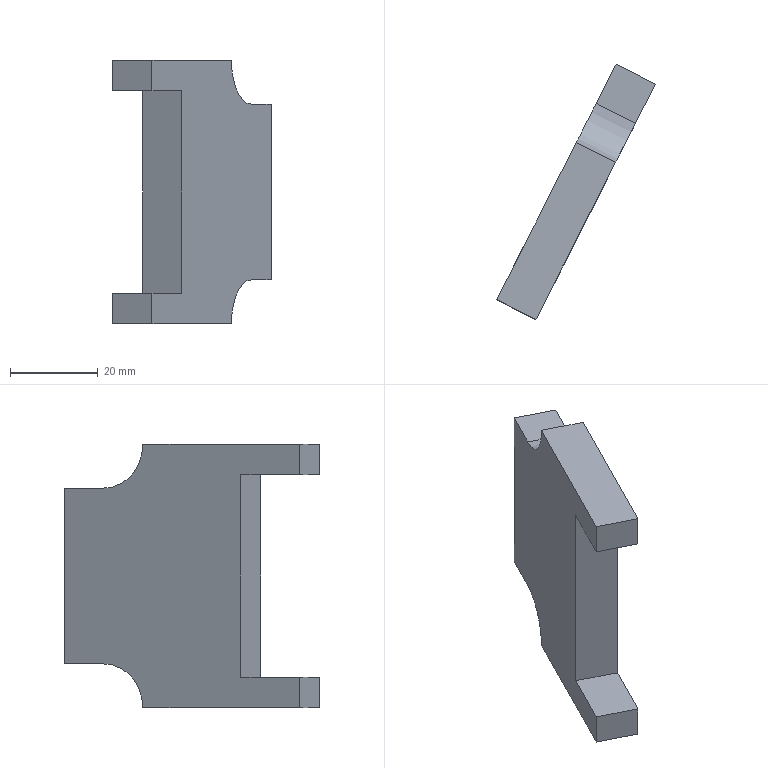Component | SolidWorks | PartThree-1 | 1 solid | 14 faces | box 36.05 x 58.04 x 60 mm | volume 25529 mm3 | plane 12 | cylinder 2 | commonest cylinder face diameters 20 x2
STEP:
#1=CARTESIAN_POINT('',(-56.846,-10.874,42.676));
#2=VERTEX_POINT('',#1);
#3=CARTESIAN_POINT('',(-56.495,-11.052,42.676));
#4=VERTEX_POINT('',#3);
#5=CARTESIAN_POINT('',(-56.846,-10.874,42.676));
#6=DIRECTION('',(0.892,-0.4521,-0.));
#7=VECTOR('',#6,39.37);
#8=LINE('',#5,#7);
#9=EDGE_CURVE('',#2,#4,#8,.T.);
#10=ORIENTED_EDGE('',*,*,#9,.F.);
#11=CARTESIAN_POINT('',(-57.024,-11.225,43.07));
#12=VERTEX_POINT('',#11);
#13=CARTESIAN_POINT('',(-56.846,-10.874,43.07));
#14=DIRECTION('',(-0.892,0.4521,0.));
#15=DIRECTION('',(-0.,-0.,1.));
#16=AXIS2_PLACEMENT_3D('',#13,#14,#15);
#17=CIRCLE('',#16,0.3937);
#18=EDGE_CURVE('',#2,#12,#17,.T.);
#19=ORIENTED_EDGE('',*,*,#18,.T.);
#20=CARTESIAN_POINT('',(-56.673,-11.403,43.07));
#21=VERTEX_POINT('',#20);
#22=CARTESIAN_POINT('',(-57.024,-11.225,43.07));
#23=DIRECTION('',(0.892,-0.4521,-0.));
#24=VECTOR('',#23,39.37);
#25=LINE('',#22,#24);
#26=EDGE_CURVE('',#12,#21,#25,.T.);
#27=ORIENTED_EDGE('',*,*,#26,.T.);
#28=CARTESIAN_POINT('',(-56.495,-11.052,43.07));
#29=DIRECTION('',(0.892,-0.4521,-0.));
#30=DIRECTION('',(-0.,-0.,1.));
#31=AXIS2_PLACEMENT_3D('',#28,#29,#30);
#32=CIRCLE('',#31,0.3937);
#33=EDGE_CURVE('',#21,#4,#32,.T.);
#34=ORIENTED_EDGE('',*,*,#33,.T.);
#35=EDGE_LOOP('',(#10,#19,#27,#34));
#36=FACE_OUTER_BOUND('',#35,.T.);
#37=CARTESIAN_POINT('',(-56.846,-10.874,43.07));
#38=DIRECTION('',(-0.892,0.4521,0.));
#39=DIRECTION('',(-0.,-0.,1.));
#40=AXIS2_PLACEMENT_3D('',#37,#38,#39);
#41=CYLINDRICAL_SURFACE('',#40,0.3937);
#42=ADVANCED_FACE('',(#36),#41,.F.);
#43=CARTESIAN_POINT('',(-56.495,-11.052,41.101));
#44=VERTEX_POINT('',#43);
#45=CARTESIAN_POINT('',(-56.846,-10.874,41.101));
#46=VERTEX_POINT('',#45);
#47=CARTESIAN_POINT('',(-56.846,-10.874,41.101));
#48=DIRECTION('',(-0.892,0.4521,0.));
#49=VECTOR('',#48,39.37);
#50=LINE('',#47,#49);
#51=EDGE_CURVE('',#44,#46,#50,.T.);
#52=ORIENTED_EDGE('',*,*,#51,.F.);
#53=CARTESIAN_POINT('',(-56.673,-11.403,40.708));
#54=VERTEX_POINT('',#53);
#55=CARTESIAN_POINT('',(-56.495,-11.052,40.708));
#56=DIRECTION('',(0.892,-0.4521,-0.));
#57=DIRECTION('',(-0.,-0.,1.));
#58=AXIS2_PLACEMENT_3D('',#55,#56,#57);
#59=CIRCLE('',#58,0.3937);
#60=EDGE_CURVE('',#44,#54,#59,.T.);
#61=ORIENTED_EDGE('',*,*,#60,.T.);
#62=CARTESIAN_POINT('',(-57.024,-11.225,40.708));
#63=VERTEX_POINT('',#62);
#64=CARTESIAN_POINT('',(-57.024,-11.225,40.708));
#65=DIRECTION('',(0.892,-0.4521,-0.));
#66=VECTOR('',#65,39.37);
#67=LINE('',#64,#66);
#68=EDGE_CURVE('',#63,#54,#67,.T.);
#69=ORIENTED_EDGE('',*,*,#68,.F.);
#70=CARTESIAN_POINT('',(-56.846,-10.874,40.708));
#71=DIRECTION('',(-0.892,0.4521,0.));
#72=DIRECTION('',(-0.,-0.,1.));
#73=AXIS2_PLACEMENT_3D('',#70,#71,#72);
#74=CIRCLE('',#73,0.3937);
#75=EDGE_CURVE('',#63,#46,#74,.T.);
#76=ORIENTED_EDGE('',*,*,#75,.T.);
#77=EDGE_LOOP('',(#52,#61,#69,#76));
#78=FACE_OUTER_BOUND('',#77,.T.);
#79=CARTESIAN_POINT('',(-56.846,-10.874,40.708));
#80=DIRECTION('',(0.892,-0.4521,-0.));
#81=DIRECTION('',(0.,0.,-1.));
#82=AXIS2_PLACEMENT_3D('',#79,#80,#81);
#83=CYLINDRICAL_SURFACE('',#82,0.3937);
#84=ADVANCED_FACE('',(#78),#83,.F.);
#85=CARTESIAN_POINT('',(-57.385,-12.808,40.708));
#86=VERTEX_POINT('',#85);
#87=CARTESIAN_POINT('',(-56.673,-11.403,40.708));
#88=DIRECTION('',(-0.4521,-0.892,-0.));
#89=VECTOR('',#88,39.37);
#90=LINE('',#87,#89);
#91=EDGE_CURVE('',#54,#86,#90,.T.);
#92=ORIENTED_EDGE('',*,*,#91,.T.);
#93=CARTESIAN_POINT('',(-57.736,-12.63,40.708));
#94=VERTEX_POINT('',#93);
#95=CARTESIAN_POINT('',(-57.736,-12.63,40.708));
#96=DIRECTION('',(0.892,-0.4521,-0.));
#97=VECTOR('',#96,39.37);
#98=LINE('',#95,#97);
#99=EDGE_CURVE('',#94,#86,#98,.T.);
#100=ORIENTED_EDGE('',*,*,#99,.F.);
#101=CARTESIAN_POINT('',(-57.024,-11.225,40.708));
#102=DIRECTION('',(-0.4521,-0.892,-0.));
#103=VECTOR('',#102,39.37);
#104=LINE('',#101,#103);
#105=EDGE_CURVE('',#63,#94,#104,.T.);
#106=ORIENTED_EDGE('',*,*,#105,.F.);
#107=ORIENTED_EDGE('',*,*,#68,.T.);
#108=EDGE_LOOP('',(#92,#100,#106,#107));
#109=FACE_OUTER_BOUND('',#108,.T.);
#110=CARTESIAN_POINT('',(-57.024,-11.225,40.708));
#111=DIRECTION('',(-0.,-0.,1.));
#112=DIRECTION('',(0.4521,0.892,0.));
#113=AXIS2_PLACEMENT_3D('',#110,#111,#112);
#114=PLANE('',#113);
#115=ADVANCED_FACE('',(#109),#114,.F.);
#116=CARTESIAN_POINT('',(-57.385,-12.808,40.983));
#117=VERTEX_POINT('',#116);
#118=CARTESIAN_POINT('',(-57.385,-12.808,40.708));
#119=DIRECTION('',(-0.,-0.,1.));
#120=VECTOR('',#119,39.37);
#121=LINE('',#118,#120);
#122=EDGE_CURVE('',#86,#117,#121,.T.);
#123=ORIENTED_EDGE('',*,*,#122,.T.);
#124=CARTESIAN_POINT('',(-57.736,-12.63,40.983));
#125=VERTEX_POINT('',#124);
#126=CARTESIAN_POINT('',(-57.736,-12.63,40.983));
#127=DIRECTION('',(0.892,-0.4521,-0.));
#128=VECTOR('',#127,39.37);
#129=LINE('',#126,#128);
#130=EDGE_CURVE('',#125,#117,#129,.T.);
#131=ORIENTED_EDGE('',*,*,#130,.F.);
#132=CARTESIAN_POINT('',(-57.736,-12.63,40.708));
#133=DIRECTION('',(-0.,-0.,1.));
#134=VECTOR('',#133,39.37);
#135=LINE('',#132,#134);
#136=EDGE_CURVE('',#94,#125,#135,.T.);
#137=ORIENTED_EDGE('',*,*,#136,.F.);
#138=ORIENTED_EDGE('',*,*,#99,.T.);
#139=EDGE_LOOP('',(#123,#131,#137,#138));
#140=FACE_OUTER_BOUND('',#139,.T.);
#141=CARTESIAN_POINT('',(-57.736,-12.63,40.708));
#142=DIRECTION('',(0.4521,0.892,0.));
#143=DIRECTION('',(-0.892,0.4521,0.));
#144=AXIS2_PLACEMENT_3D('',#141,#142,#143);
#145=PLANE('',#144);
#146=ADVANCED_FACE('',(#140),#145,.F.);
#147=CARTESIAN_POINT('',(-57.118,-12.281,40.983));
#148=VERTEX_POINT('',#147);
#149=CARTESIAN_POINT('',(-57.385,-12.808,40.983));
#150=DIRECTION('',(0.4521,0.892,0.));
#151=VECTOR('',#150,39.37);
#152=LINE('',#149,#151);
#153=EDGE_CURVE('',#117,#148,#152,.T.);
#154=ORIENTED_EDGE('',*,*,#153,.T.);
#155=CARTESIAN_POINT('',(-57.469,-12.103,40.983));
#156=VERTEX_POINT('',#155);
#157=CARTESIAN_POINT('',(-57.469,-12.103,40.983));
#158=DIRECTION('',(0.892,-0.4521,-0.));
#159=VECTOR('',#158,39.37);
#160=LINE('',#157,#159);
#161=EDGE_CURVE('',#156,#148,#160,.T.);
#162=ORIENTED_EDGE('',*,*,#161,.F.);
#163=CARTESIAN_POINT('',(-57.736,-12.63,40.983));
#164=DIRECTION('',(0.4521,0.892,0.));
#165=VECTOR('',#164,39.37);
#166=LINE('',#163,#165);
#167=EDGE_CURVE('',#125,#156,#166,.T.);
#168=ORIENTED_EDGE('',*,*,#167,.F.);
#169=ORIENTED_EDGE('',*,*,#130,.T.);
#170=EDGE_LOOP('',(#154,#162,#168,#169));
#171=FACE_OUTER_BOUND('',#170,.T.);
#172=CARTESIAN_POINT('',(-57.736,-12.63,40.983));
#173=DIRECTION('',(0.,0.,-1.));
#174=DIRECTION('',(-0.892,0.4521,0.));
#175=AXIS2_PLACEMENT_3D('',#172,#173,#174);
#176=PLANE('',#175);
#177=ADVANCED_FACE('',(#171),#176,.F.);
#178=CARTESIAN_POINT('',(-57.118,-12.281,42.794));
#179=VERTEX_POINT('',#178);
#180=CARTESIAN_POINT('',(-57.118,-12.281,42.794));
#181=DIRECTION('',(0.,0.,-1.));
#182=VECTOR('',#181,39.37);
#183=LINE('',#180,#182);
#184=EDGE_CURVE('',#179,#148,#183,.T.);
#185=ORIENTED_EDGE('',*,*,#184,.F.);
#186=CARTESIAN_POINT('',(-57.469,-12.103,42.794));
#187=VERTEX_POINT('',#186);
#188=CARTESIAN_POINT('',(-57.469,-12.103,42.794));
#189=DIRECTION('',(0.892,-0.4521,-0.));
#190=VECTOR('',#189,39.37);
#191=LINE('',#188,#190);
#192=EDGE_CURVE('',#187,#179,#191,.T.);
#193=ORIENTED_EDGE('',*,*,#192,.F.);
#194=CARTESIAN_POINT('',(-57.469,-12.103,42.794));
#195=DIRECTION('',(0.,0.,-1.));
#196=VECTOR('',#195,39.37);
#197=LINE('',#194,#196);
#198=EDGE_CURVE('',#187,#156,#197,.T.);
#199=ORIENTED_EDGE('',*,*,#198,.T.);
#200=ORIENTED_EDGE('',*,*,#161,.T.);
#201=EDGE_LOOP('',(#185,#193,#199,#200));
#202=FACE_OUTER_BOUND('',#201,.T.);
#203=CARTESIAN_POINT('',(-57.469,-12.103,42.794));
#204=DIRECTION('',(-0.4521,-0.892,-0.));
#205=DIRECTION('',(0.892,-0.4521,-0.));
#206=AXIS2_PLACEMENT_3D('',#203,#204,#205);
#207=PLANE('',#206);
#208=ADVANCED_FACE('',(#202),#207,.T.);
#209=CARTESIAN_POINT('',(-57.385,-12.808,42.794));
#210=VERTEX_POINT('',#209);
#211=CARTESIAN_POINT('',(-57.385,-12.808,42.794));
#212=DIRECTION('',(0.4521,0.892,0.));
#213=VECTOR('',#212,39.37);
#214=LINE('',#211,#213);
#215=EDGE_CURVE('',#210,#179,#214,.T.);
#216=ORIENTED_EDGE('',*,*,#215,.F.);
#217=CARTESIAN_POINT('',(-57.736,-12.63,42.794));
#218=VERTEX_POINT('',#217);
#219=CARTESIAN_POINT('',(-57.736,-12.63,42.794));
#220=DIRECTION('',(0.892,-0.4521,-0.));
#221=VECTOR('',#220,39.37);
#222=LINE('',#219,#221);
#223=EDGE_CURVE('',#218,#210,#222,.T.);
#224=ORIENTED_EDGE('',*,*,#223,.F.);
#225=CARTESIAN_POINT('',(-57.736,-12.63,42.794));
#226=DIRECTION('',(0.4521,0.892,0.));
#227=VECTOR('',#226,39.37);
#228=LINE('',#225,#227);
#229=EDGE_CURVE('',#218,#187,#228,.T.);
#230=ORIENTED_EDGE('',*,*,#229,.T.);
#231=ORIENTED_EDGE('',*,*,#192,.T.);
#232=EDGE_LOOP('',(#216,#224,#230,#231));
#233=FACE_OUTER_BOUND('',#232,.T.);
#234=CARTESIAN_POINT('',(-57.736,-12.63,42.794));
#235=DIRECTION('',(0.,0.,-1.));
#236=DIRECTION('',(-0.892,0.4521,0.));
#237=AXIS2_PLACEMENT_3D('',#234,#235,#236);
#238=PLANE('',#237);
#239=ADVANCED_FACE('',(#233),#238,.T.);
#240=CARTESIAN_POINT('',(-57.385,-12.808,43.07));
#241=VERTEX_POINT('',#240);
#242=CARTESIAN_POINT('',(-57.385,-12.808,43.07));
#243=DIRECTION('',(0.,0.,-1.));
#244=VECTOR('',#243,39.37);
#245=LINE('',#242,#244);
#246=EDGE_CURVE('',#241,#210,#245,.T.);
#247=ORIENTED_EDGE('',*,*,#246,.F.);
#248=CARTESIAN_POINT('',(-57.736,-12.63,43.07));
#249=VERTEX_POINT('',#248);
#250=CARTESIAN_POINT('',(-57.736,-12.63,43.07));
#251=DIRECTION('',(0.892,-0.4521,-0.));
#252=VECTOR('',#251,39.37);
#253=LINE('',#250,#252);
#254=EDGE_CURVE('',#249,#241,#253,.T.);
#255=ORIENTED_EDGE('',*,*,#254,.F.);
#256=CARTESIAN_POINT('',(-57.736,-12.63,43.07));
#257=DIRECTION('',(0.,0.,-1.));
#258=VECTOR('',#257,39.37);
#259=LINE('',#256,#258);
#260=EDGE_CURVE('',#249,#218,#259,.T.);
#261=ORIENTED_EDGE('',*,*,#260,.T.);
#262=ORIENTED_EDGE('',*,*,#223,.T.);
#263=EDGE_LOOP('',(#247,#255,#261,#262));
#264=FACE_OUTER_BOUND('',#263,.T.);
#265=CARTESIAN_POINT('',(-57.736,-12.63,43.07));
#266=DIRECTION('',(-0.4521,-0.892,-0.));
#267=DIRECTION('',(0.892,-0.4521,-0.));
#268=AXIS2_PLACEMENT_3D('',#265,#266,#267);
#269=PLANE('',#268);
#270=ADVANCED_FACE('',(#264),#269,.T.);
#271=CARTESIAN_POINT('',(-56.673,-11.403,43.07));
#272=DIRECTION('',(-0.4521,-0.892,-0.));
#273=VECTOR('',#272,39.37);
#274=LINE('',#271,#273);
#275=EDGE_CURVE('',#21,#241,#274,.T.);
#276=ORIENTED_EDGE('',*,*,#275,.F.);
#277=ORIENTED_EDGE('',*,*,#26,.F.);
#278=CARTESIAN_POINT('',(-57.024,-11.225,43.07));
#279=DIRECTION('',(-0.4521,-0.892,-0.));
#280=VECTOR('',#279,39.37);
#281=LINE('',#278,#280);
#282=EDGE_CURVE('',#12,#249,#281,.T.);
#283=ORIENTED_EDGE('',*,*,#282,.T.);
#284=ORIENTED_EDGE('',*,*,#254,.T.);
#285=EDGE_LOOP('',(#276,#277,#283,#284));
#286=FACE_OUTER_BOUND('',#285,.T.);
#287=CARTESIAN_POINT('',(-57.024,-11.225,43.07));
#288=DIRECTION('',(-0.,-0.,1.));
#289=DIRECTION('',(0.4521,0.892,0.));
#290=AXIS2_PLACEMENT_3D('',#287,#288,#289);
#291=PLANE('',#290);
#292=ADVANCED_FACE('',(#286),#291,.T.);
#293=CARTESIAN_POINT('',(-56.668,-10.523,42.676));
#294=VERTEX_POINT('',#293);
#295=CARTESIAN_POINT('',(-56.668,-10.523,42.676));
#296=DIRECTION('',(-0.4521,-0.892,-0.));
#297=VECTOR('',#296,39.37);
#298=LINE('',#295,#297);
#299=EDGE_CURVE('',#294,#2,#298,.T.);
#300=ORIENTED_EDGE('',*,*,#299,.T.);
#301=ORIENTED_EDGE('',*,*,#9,.T.);
#302=CARTESIAN_POINT('',(-56.317,-10.701,42.676));
#303=VERTEX_POINT('',#302);
#304=CARTESIAN_POINT('',(-56.317,-10.701,42.676));
#305=DIRECTION('',(-0.4521,-0.892,-0.));
#306=VECTOR('',#305,39.37);
#307=LINE('',#304,#306);
#308=EDGE_CURVE('',#303,#4,#307,.T.);
#309=ORIENTED_EDGE('',*,*,#308,.F.);
#310=CARTESIAN_POINT('',(-56.668,-10.523,42.676));
#311=DIRECTION('',(0.892,-0.4521,-0.));
#312=VECTOR('',#311,39.37);
#313=LINE('',#310,#312);
#314=EDGE_CURVE('',#294,#303,#313,.T.);
#315=ORIENTED_EDGE('',*,*,#314,.F.);
#316=EDGE_LOOP('',(#300,#301,#309,#315));
#317=FACE_OUTER_BOUND('',#316,.T.);
#318=CARTESIAN_POINT('',(-56.668,-10.523,42.676));
#319=DIRECTION('',(-0.,-0.,1.));
#320=DIRECTION('',(0.892,-0.4521,-0.));
#321=AXIS2_PLACEMENT_3D('',#318,#319,#320);
#322=PLANE('',#321);
#323=ADVANCED_FACE('',(#317),#322,.T.);
#324=CARTESIAN_POINT('',(-56.317,-10.701,41.101));
#325=VERTEX_POINT('',#324);
#326=CARTESIAN_POINT('',(-56.317,-10.701,41.101));
#327=DIRECTION('',(-0.,-0.,1.));
#328=VECTOR('',#327,39.37);
#329=LINE('',#326,#328);
#330=EDGE_CURVE('',#325,#303,#329,.T.);
#331=ORIENTED_EDGE('',*,*,#330,.F.);
#332=CARTESIAN_POINT('',(-56.668,-10.523,41.101));
#333=VERTEX_POINT('',#332);
#334=CARTESIAN_POINT('',(-56.668,-10.523,41.101));
#335=DIRECTION('',(0.892,-0.4521,-0.));
#336=VECTOR('',#335,39.37);
#337=LINE('',#334,#336);
#338=EDGE_CURVE('',#333,#325,#337,.T.);
#339=ORIENTED_EDGE('',*,*,#338,.F.);
#340=CARTESIAN_POINT('',(-56.668,-10.523,41.101));
#341=DIRECTION('',(-0.,-0.,1.));
#342=VECTOR('',#341,39.37);
#343=LINE('',#340,#342);
#344=EDGE_CURVE('',#333,#294,#343,.T.);
#345=ORIENTED_EDGE('',*,*,#344,.T.);
#346=ORIENTED_EDGE('',*,*,#314,.T.);
#347=EDGE_LOOP('',(#331,#339,#345,#346));
#348=FACE_OUTER_BOUND('',#347,.T.);
#349=CARTESIAN_POINT('',(-56.668,-10.523,41.101));
#350=DIRECTION('',(0.4521,0.892,0.));
#351=DIRECTION('',(-0.892,0.4521,0.));
#352=AXIS2_PLACEMENT_3D('',#349,#350,#351);
#353=PLANE('',#352);
#354=ADVANCED_FACE('',(#348),#353,.T.);
#355=CARTESIAN_POINT('',(-56.317,-10.701,41.101));
#356=DIRECTION('',(-0.4521,-0.892,-0.));
#357=VECTOR('',#356,39.37);
#358=LINE('',#355,#357);
#359=EDGE_CURVE('',#325,#44,#358,.T.);
#360=ORIENTED_EDGE('',*,*,#359,.T.);
#361=ORIENTED_EDGE('',*,*,#51,.T.);
#362=CARTESIAN_POINT('',(-56.668,-10.523,41.101));
#363=DIRECTION('',(-0.4521,-0.892,-0.));
#364=VECTOR('',#363,39.37);
#365=LINE('',#362,#364);
#366=EDGE_CURVE('',#333,#46,#365,.T.);
#367=ORIENTED_EDGE('',*,*,#366,.F.);
#368=ORIENTED_EDGE('',*,*,#338,.T.);
#369=EDGE_LOOP('',(#360,#361,#367,#368));
#370=FACE_OUTER_BOUND('',#369,.T.);
#371=CARTESIAN_POINT('',(-56.668,-10.523,41.101));
#372=DIRECTION('',(-0.,-0.,1.));
#373=DIRECTION('',(0.892,-0.4521,-0.));
#374=AXIS2_PLACEMENT_3D('',#371,#372,#373);
#375=PLANE('',#374);
#376=ADVANCED_FACE('',(#370),#375,.F.);
#377=ORIENTED_EDGE('',*,*,#75,.F.);
#378=ORIENTED_EDGE('',*,*,#105,.T.);
#379=ORIENTED_EDGE('',*,*,#136,.T.);
#380=ORIENTED_EDGE('',*,*,#167,.T.);
#381=ORIENTED_EDGE('',*,*,#198,.F.);
#382=ORIENTED_EDGE('',*,*,#229,.F.);
#383=ORIENTED_EDGE('',*,*,#260,.F.);
#384=ORIENTED_EDGE('',*,*,#282,.F.);
#385=ORIENTED_EDGE('',*,*,#18,.F.);
#386=ORIENTED_EDGE('',*,*,#299,.F.);
#387=ORIENTED_EDGE('',*,*,#344,.F.);
#388=ORIENTED_EDGE('',*,*,#366,.T.);
#389=EDGE_LOOP('',(#377,#378,#379,#380,#381,#382,#383,#384,#385,#386,#387,#388));
#390=FACE_OUTER_BOUND('',#389,.T.);
#391=CARTESIAN_POINT('',(-57.42,-12.006,42.103));
#392=DIRECTION('',(-0.892,0.4521,0.));
#393=DIRECTION('',(-0.,-0.,1.));
#394=AXIS2_PLACEMENT_3D('',#391,#392,#393);
#395=PLANE('',#394);
#396=ADVANCED_FACE('',(#390),#395,.T.);
#397=ORIENTED_EDGE('',*,*,#33,.F.);
#398=ORIENTED_EDGE('',*,*,#275,.T.);
#399=ORIENTED_EDGE('',*,*,#246,.T.);
#400=ORIENTED_EDGE('',*,*,#215,.T.);
#401=ORIENTED_EDGE('',*,*,#184,.T.);
#402=ORIENTED_EDGE('',*,*,#153,.F.);
#403=ORIENTED_EDGE('',*,*,#122,.F.);
#404=ORIENTED_EDGE('',*,*,#91,.F.);
#405=ORIENTED_EDGE('',*,*,#60,.F.);
#406=ORIENTED_EDGE('',*,*,#359,.F.);
#407=ORIENTED_EDGE('',*,*,#330,.T.);
#408=ORIENTED_EDGE('',*,*,#308,.T.);
#409=EDGE_LOOP('',(#397,#398,#399,#400,#401,#402,#403,#404,#405,#406,#407,#408));
#410=FACE_OUTER_BOUND('',#409,.T.);
#411=CARTESIAN_POINT('',(-57.069,-12.184,42.103));
#412=DIRECTION('',(-0.892,0.4521,0.));
#413=DIRECTION('',(-0.,-0.,1.));
#414=AXIS2_PLACEMENT_3D('',#411,#412,#413);
#415=PLANE('',#414);
#416=ADVANCED_FACE('',(#410),#415,.F.);
#417=CLOSED_SHELL('',(#42,#84,#115,#146,#177,#208,#239,#270,#292,#323,#354,#376,#396,#416));
#418=MANIFOLD_SOLID_BREP('',#417);
#419=CARTESIAN_POINT('',(0.,0.,0.));
#420=DIRECTION('',(0.,0.,1.));
#421=DIRECTION('',(1.,0.,0.));
#422=AXIS2_PLACEMENT_3D('',#419,#420,#421);
#423=(LENGTH_UNIT()NAMED_UNIT(*)SI_UNIT($,.METRE.));
#424=LENGTH_MEASURE_WITH_UNIT(LENGTH_MEASURE(0.0254),#423);
#425=DIMENSIONAL_EXPONENTS(1.,0.,0.,0.,0.,0.,0.);
#426=(CONVERSION_BASED_UNIT('',#424)LENGTH_UNIT()NAMED_UNIT(#425));
#427=UNCERTAINTY_MEASURE_WITH_UNIT(LENGTH_MEASURE(0.00001),#426,'','');
#428=(NAMED_UNIT(*)PLANE_ANGLE_UNIT()SI_UNIT($,.RADIAN.));
#429=(NAMED_UNIT(*)SI_UNIT($,.STERADIAN.)SOLID_ANGLE_UNIT());
#430=(GEOMETRIC_REPRESENTATION_CONTEXT(3)GLOBAL_UNCERTAINTY_ASSIGNED_CONTEXT((#427))GLOBAL_UNIT_ASSIGNED_CONTEXT((#426,#428,#429))REPRESENTATION_CONTEXT('',''));
#431=ADVANCED_BREP_SHAPE_REPRESENTATION('',(#418,#422),#430);
#432=COLOUR_RGB('',0.7922,0.8196,0.9333);
#433=FILL_AREA_STYLE_COLOUR('',#432);
#434=FILL_AREA_STYLE('',(#433));
#435=SURFACE_STYLE_FILL_AREA(#434);
#436=SURFACE_SIDE_STYLE('',(#435));
#437=SURFACE_STYLE_USAGE(.BOTH.,#436);
#438=PRESENTATION_STYLE_ASSIGNMENT((#437));
#439=STYLED_ITEM('',(#438),#418);
#440=PRESENTATION_LAYER_ASSIGNMENT('','',(#439));
#441=(LENGTH_UNIT()NAMED_UNIT(*)SI_UNIT($,.METRE.));
#442=LENGTH_MEASURE_WITH_UNIT(LENGTH_MEASURE(0.0254),#441);
#443=DIMENSIONAL_EXPONENTS(1.,0.,0.,0.,0.,0.,0.);
#444=(CONVERSION_BASED_UNIT('',#442)LENGTH_UNIT()NAMED_UNIT(#443));
#445=UNCERTAINTY_MEASURE_WITH_UNIT(LENGTH_MEASURE(0.00001),#444,'','');
#446=(NAMED_UNIT(*)PLANE_ANGLE_UNIT()SI_UNIT($,.RADIAN.));
#447=(NAMED_UNIT(*)SI_UNIT($,.STERADIAN.)SOLID_ANGLE_UNIT());
#448=(GEOMETRIC_REPRESENTATION_CONTEXT(3)GLOBAL_UNCERTAINTY_ASSIGNED_CONTEXT((#445))GLOBAL_UNIT_ASSIGNED_CONTEXT((#444,#446,#447))REPRESENTATION_CONTEXT('',''));
#449=MECHANICAL_DESIGN_GEOMETRIC_PRESENTATION_REPRESENTATION('',(#439),#448);